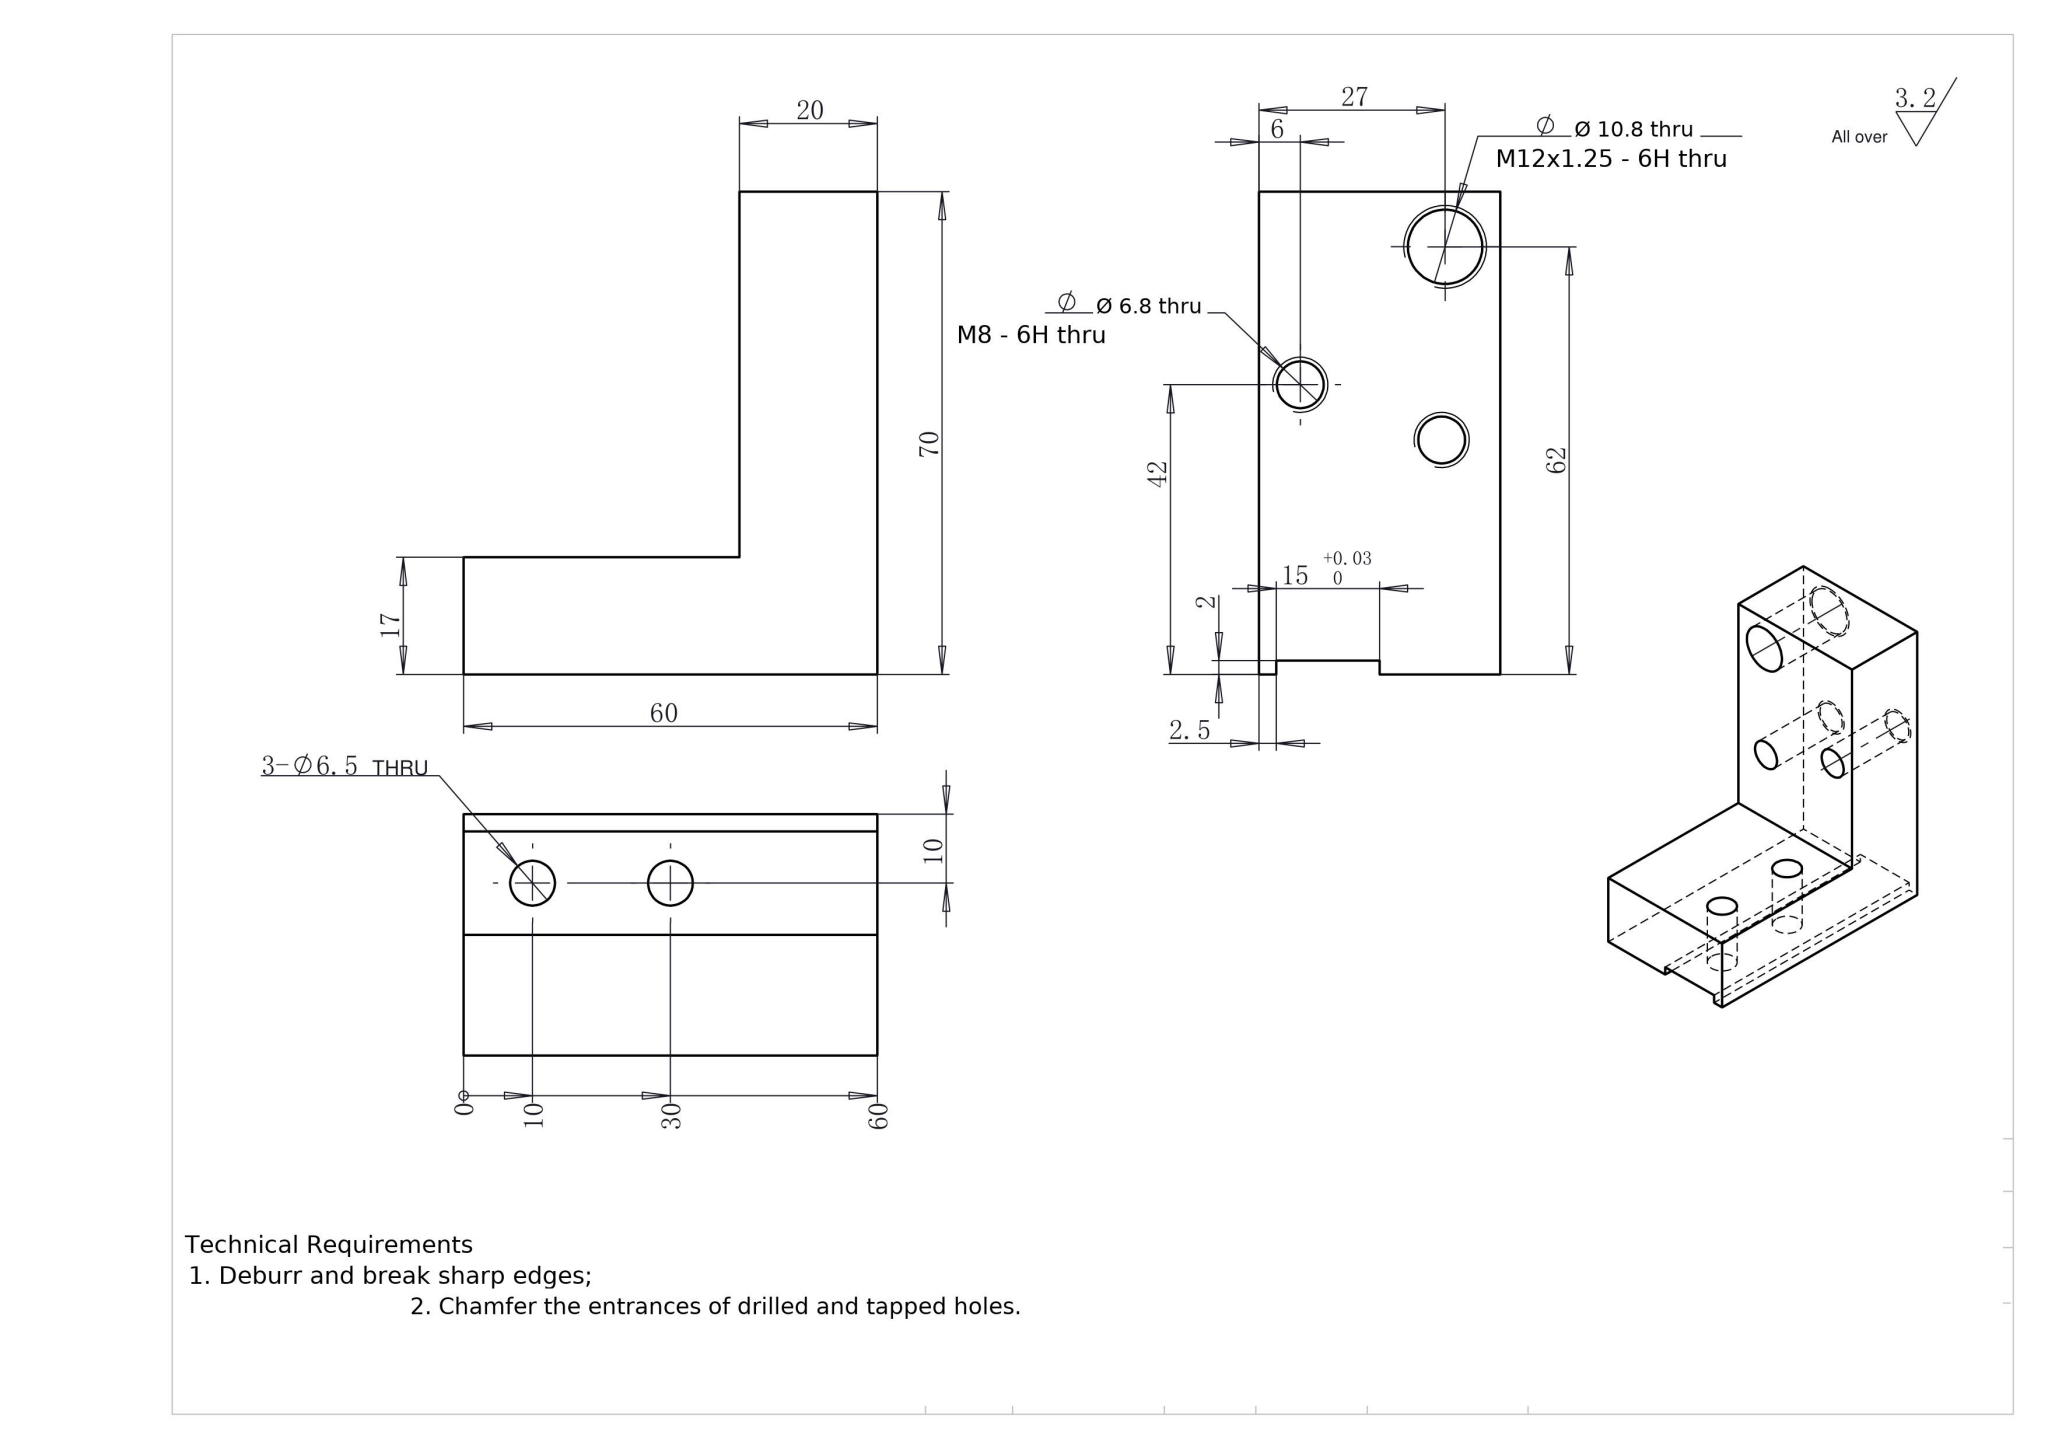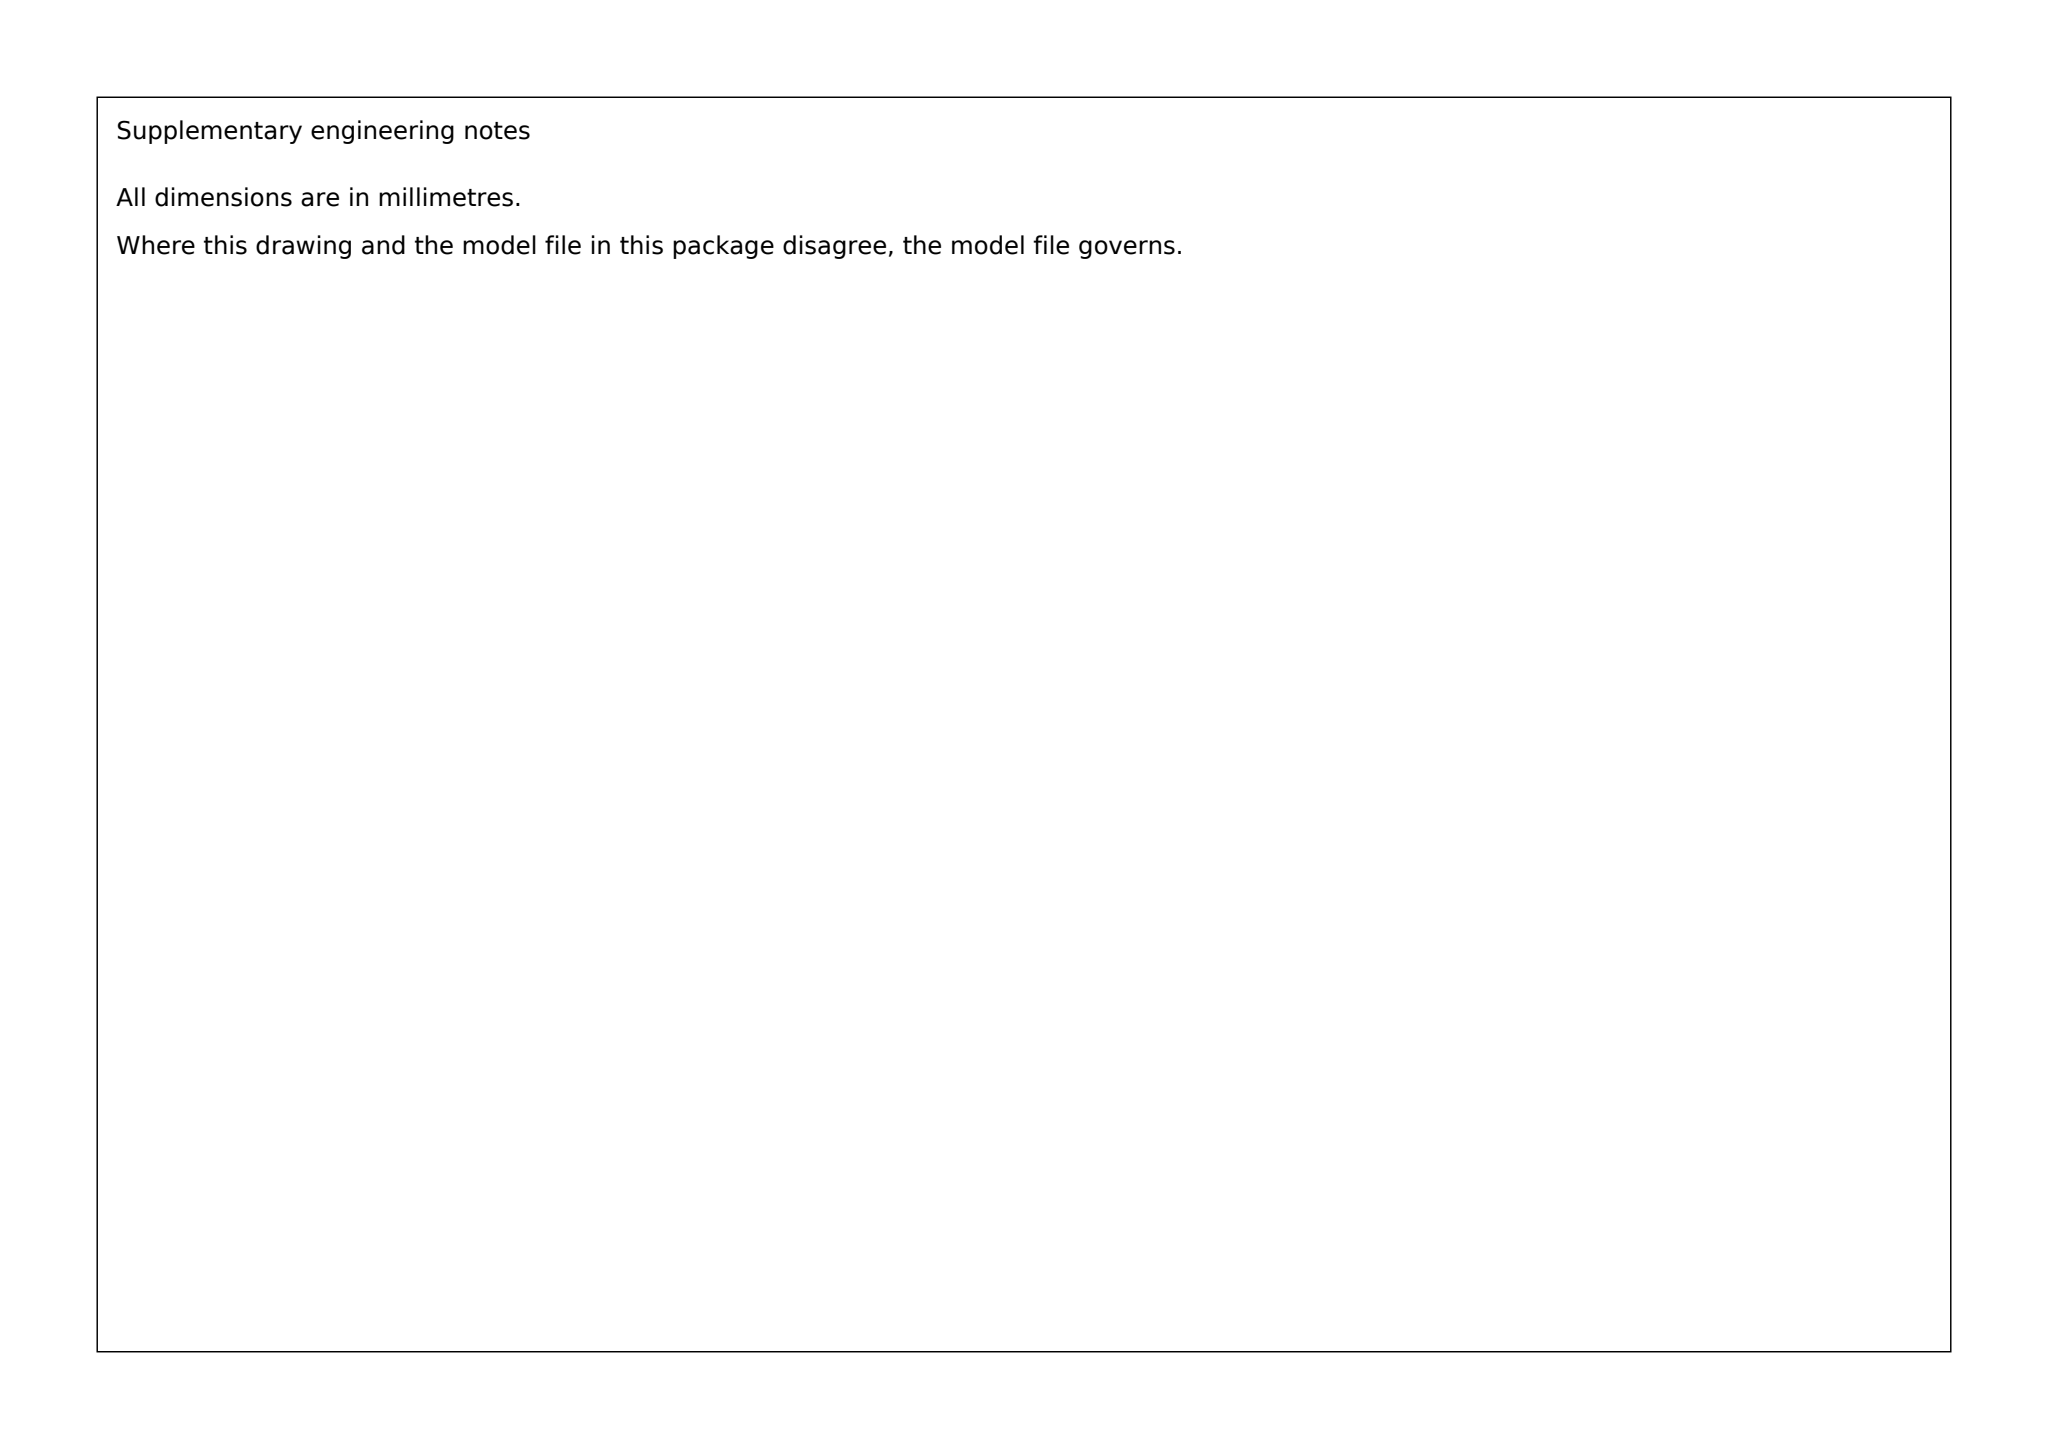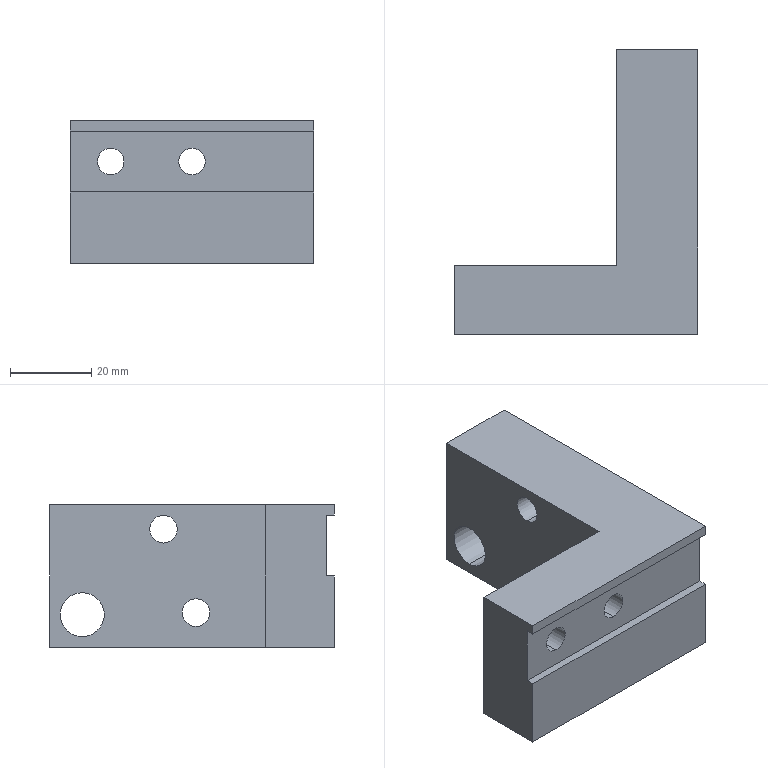Part | SolidWorks | mm | 1 solid | 22 faces | box 60 x 70 x 35 mm | volume 66720 mm3 | plane 12 | cylinder 10 | commonest cylinder face diameters 6.8 x4 6.5 x4 10.8 x2
build123d program:
from build123d import *

# Parameters (mm, degrees)
BOSS_EXTRUDE1_DEPTH     = 35
SKETCH2_W               = 15
SKETCH2_H               = 2
CUT_EXTRUDE1_DEPTH      = 99.615
SKETCH3_R               = 3.25
CUT_EXTRUDE2_DEPTH      = 98.206
M8_TAPPED_HOLE2_D       = 6.8
M12X1_25_TAPPED_HOLE1_D = 10.8
M8_TAPPED_HOLE1_D       = 6.8


with BuildPart() as part:
    # Sketch1 → Boss-Extrude1 (new body)
    with BuildSketch(Plane.XY):
        Polygon((40, 70), (40, 17), (0, 17), (0, 0), (60, 0), (60, 70), align=None)
    extrude(amount=-BOSS_EXTRUDE1_DEPTH)

    # Sketch2 → Cut-Extrude1 (cut, through all)
    with BuildSketch(Plane(origin=(60, 0, 0), x_dir=(0, 0, -1), z_dir=(1, 0, 0))):
        with Locations((10, 1)):
            Rectangle(SKETCH2_W, SKETCH2_H)
    extrude(amount=-CUT_EXTRUDE1_DEPTH, mode=Mode.SUBTRACT)

    # Sketch3 → Cut-Extrude2 (cut, through all)
    with BuildSketch(Plane.XZ.offset(-2)):
        with Locations(Location((10, -10, 0), (0, 0, 270))):
            Circle(SKETCH3_R)
        with Locations(Location((30, -10, 0), (0, 0, 270))):
            Circle(SKETCH3_R)
    extrude(amount=-CUT_EXTRUDE2_DEPTH, mode=Mode.SUBTRACT)

    # M8 Tapped Hole2 (through all)
    with Locations(Plane(origin=(60, 0, 0), x_dir=(0, 0, -1), z_dir=(1, 0, 0))):
        with Locations((6, 42)):
            Hole(M8_TAPPED_HOLE2_D / 2)

    # M12x1.25 Tapped Hole1 (through all)
    with Locations(Plane(origin=(60, 0, 0), x_dir=(0, 0, -1), z_dir=(1, 0, 0))):
        with Locations((27, 62)):
            Hole(M12X1_25_TAPPED_HOLE1_D / 2)

    # M8 Tapped Hole1 (through all)
    with Locations(Plane(origin=(60, 0, 0), x_dir=(0, 0, -1), z_dir=(1, 0, 0))):
        with Locations((26.5, 34)):
            Hole(M8_TAPPED_HOLE1_D / 2)


solid = part.part
STEP:
#1=CARTESIAN_POINT('',(40.,34.,-29.9));
#2=VERTEX_POINT('',#1);
#3=CARTESIAN_POINT('',(40.,34.,-23.1));
#4=VERTEX_POINT('',#3);
#5=CARTESIAN_POINT('',(40.,34.,-26.5));
#6=DIRECTION('',(-1.,0.,0.));
#7=DIRECTION('',(-0.,-1.,0.));
#8=AXIS2_PLACEMENT_3D('',#5,#6,#7);
#9=CIRCLE('',#8,3.4);
#10=EDGE_CURVE('',#2,#4,#9,.T.);
#11=ORIENTED_EDGE('',*,*,#10,.T.);
#12=CARTESIAN_POINT('',(60.,34.,-23.1));
#13=VERTEX_POINT('',#12);
#14=CARTESIAN_POINT('',(60.,34.,-23.1));
#15=DIRECTION('',(1.,0.,0.));
#16=VECTOR('',#15,1000.);
#17=LINE('',#14,#16);
#18=EDGE_CURVE('',#4,#13,#17,.T.);
#19=ORIENTED_EDGE('',*,*,#18,.T.);
#20=CARTESIAN_POINT('',(60.,34.,-29.9));
#21=VERTEX_POINT('',#20);
#22=CARTESIAN_POINT('',(60.,34.,-26.5));
#23=DIRECTION('',(1.,0.,0.));
#24=DIRECTION('',(0.,0.,-1.));
#25=AXIS2_PLACEMENT_3D('',#22,#23,#24);
#26=CIRCLE('',#25,3.4);
#27=EDGE_CURVE('',#13,#21,#26,.T.);
#28=ORIENTED_EDGE('',*,*,#27,.T.);
#29=CARTESIAN_POINT('',(60.,34.,-29.9));
#30=DIRECTION('',(1.,0.,0.));
#31=VECTOR('',#30,1000.);
#32=LINE('',#29,#31);
#33=EDGE_CURVE('',#2,#21,#32,.T.);
#34=ORIENTED_EDGE('',*,*,#33,.F.);
#35=EDGE_LOOP('',(#11,#19,#28,#34));
#36=FACE_OUTER_BOUND('',#35,.T.);
#37=CARTESIAN_POINT('',(60.,34.,-26.5));
#38=DIRECTION('',(1.,0.,0.));
#39=DIRECTION('',(0.,0.,-1.));
#40=AXIS2_PLACEMENT_3D('',#37,#38,#39);
#41=CYLINDRICAL_SURFACE('',#40,3.4);
#42=ADVANCED_FACE('',(#36),#41,.F.);
#43=CARTESIAN_POINT('',(40.,62.,-32.4));
#44=VERTEX_POINT('',#43);
#45=CARTESIAN_POINT('',(40.,62.,-21.6));
#46=VERTEX_POINT('',#45);
#47=CARTESIAN_POINT('',(40.,62.,-27.));
#48=DIRECTION('',(-1.,0.,0.));
#49=DIRECTION('',(-0.,-1.,0.));
#50=AXIS2_PLACEMENT_3D('',#47,#48,#49);
#51=CIRCLE('',#50,5.4);
#52=EDGE_CURVE('',#44,#46,#51,.T.);
#53=ORIENTED_EDGE('',*,*,#52,.T.);
#54=CARTESIAN_POINT('',(60.,62.,-21.6));
#55=VERTEX_POINT('',#54);
#56=CARTESIAN_POINT('',(60.,62.,-21.6));
#57=DIRECTION('',(1.,0.,0.));
#58=VECTOR('',#57,1000.);
#59=LINE('',#56,#58);
#60=EDGE_CURVE('',#46,#55,#59,.T.);
#61=ORIENTED_EDGE('',*,*,#60,.T.);
#62=CARTESIAN_POINT('',(60.,62.,-32.4));
#63=VERTEX_POINT('',#62);
#64=CARTESIAN_POINT('',(60.,62.,-27.));
#65=DIRECTION('',(1.,0.,0.));
#66=DIRECTION('',(0.,0.,-1.));
#67=AXIS2_PLACEMENT_3D('',#64,#65,#66);
#68=CIRCLE('',#67,5.4);
#69=EDGE_CURVE('',#55,#63,#68,.T.);
#70=ORIENTED_EDGE('',*,*,#69,.T.);
#71=CARTESIAN_POINT('',(60.,62.,-32.4));
#72=DIRECTION('',(1.,0.,0.));
#73=VECTOR('',#72,1000.);
#74=LINE('',#71,#73);
#75=EDGE_CURVE('',#44,#63,#74,.T.);
#76=ORIENTED_EDGE('',*,*,#75,.F.);
#77=EDGE_LOOP('',(#53,#61,#70,#76));
#78=FACE_OUTER_BOUND('',#77,.T.);
#79=CARTESIAN_POINT('',(60.,62.,-27.));
#80=DIRECTION('',(1.,0.,0.));
#81=DIRECTION('',(0.,0.,-1.));
#82=AXIS2_PLACEMENT_3D('',#79,#80,#81);
#83=CYLINDRICAL_SURFACE('',#82,5.4);
#84=ADVANCED_FACE('',(#78),#83,.F.);
#85=CARTESIAN_POINT('',(40.,42.,-9.4));
#86=VERTEX_POINT('',#85);
#87=CARTESIAN_POINT('',(40.,42.,-2.6));
#88=VERTEX_POINT('',#87);
#89=CARTESIAN_POINT('',(40.,42.,-6.));
#90=DIRECTION('',(-1.,0.,0.));
#91=DIRECTION('',(-0.,-1.,0.));
#92=AXIS2_PLACEMENT_3D('',#89,#90,#91);
#93=CIRCLE('',#92,3.4);
#94=EDGE_CURVE('',#86,#88,#93,.T.);
#95=ORIENTED_EDGE('',*,*,#94,.T.);
#96=CARTESIAN_POINT('',(60.,42.,-2.6));
#97=VERTEX_POINT('',#96);
#98=CARTESIAN_POINT('',(60.,42.,-2.6));
#99=DIRECTION('',(1.,0.,0.));
#100=VECTOR('',#99,1000.);
#101=LINE('',#98,#100);
#102=EDGE_CURVE('',#88,#97,#101,.T.);
#103=ORIENTED_EDGE('',*,*,#102,.T.);
#104=CARTESIAN_POINT('',(60.,42.,-9.4));
#105=VERTEX_POINT('',#104);
#106=CARTESIAN_POINT('',(60.,42.,-6.));
#107=DIRECTION('',(1.,0.,0.));
#108=DIRECTION('',(0.,0.,-1.));
#109=AXIS2_PLACEMENT_3D('',#106,#107,#108);
#110=CIRCLE('',#109,3.4);
#111=EDGE_CURVE('',#97,#105,#110,.T.);
#112=ORIENTED_EDGE('',*,*,#111,.T.);
#113=CARTESIAN_POINT('',(60.,42.,-9.4));
#114=DIRECTION('',(1.,0.,0.));
#115=VECTOR('',#114,1000.);
#116=LINE('',#113,#115);
#117=EDGE_CURVE('',#86,#105,#116,.T.);
#118=ORIENTED_EDGE('',*,*,#117,.F.);
#119=EDGE_LOOP('',(#95,#103,#112,#118));
#120=FACE_OUTER_BOUND('',#119,.T.);
#121=CARTESIAN_POINT('',(60.,42.,-6.));
#122=DIRECTION('',(1.,0.,0.));
#123=DIRECTION('',(0.,0.,-1.));
#124=AXIS2_PLACEMENT_3D('',#121,#122,#123);
#125=CYLINDRICAL_SURFACE('',#124,3.4);
#126=ADVANCED_FACE('',(#120),#125,.F.);
#127=CARTESIAN_POINT('',(30.,17.,-13.25));
#128=VERTEX_POINT('',#127);
#129=CARTESIAN_POINT('',(30.,17.,-6.75));
#130=VERTEX_POINT('',#129);
#131=CARTESIAN_POINT('',(30.,17.,-10.));
#132=DIRECTION('',(0.,1.,0.));
#133=DIRECTION('',(0.,0.,1.));
#134=AXIS2_PLACEMENT_3D('',#131,#132,#133);
#135=CIRCLE('',#134,3.25);
#136=EDGE_CURVE('',#128,#130,#135,.T.);
#137=ORIENTED_EDGE('',*,*,#136,.T.);
#138=CARTESIAN_POINT('',(30.,2.,-6.75));
#139=VERTEX_POINT('',#138);
#140=CARTESIAN_POINT('',(30.,70.,-6.75));
#141=DIRECTION('',(0.,-1.,-0.));
#142=VECTOR('',#141,1000.);
#143=LINE('',#140,#142);
#144=EDGE_CURVE('',#130,#139,#143,.T.);
#145=ORIENTED_EDGE('',*,*,#144,.T.);
#146=CARTESIAN_POINT('',(30.,2.,-13.25));
#147=VERTEX_POINT('',#146);
#148=CARTESIAN_POINT('',(30.,2.,-10.));
#149=DIRECTION('',(0.,-1.,-0.));
#150=DIRECTION('',(0.,0.,-1.));
#151=AXIS2_PLACEMENT_3D('',#148,#149,#150);
#152=CIRCLE('',#151,3.25);
#153=EDGE_CURVE('',#139,#147,#152,.T.);
#154=ORIENTED_EDGE('',*,*,#153,.T.);
#155=CARTESIAN_POINT('',(30.,70.,-13.25));
#156=DIRECTION('',(0.,-1.,-0.));
#157=VECTOR('',#156,1000.);
#158=LINE('',#155,#157);
#159=EDGE_CURVE('',#128,#147,#158,.T.);
#160=ORIENTED_EDGE('',*,*,#159,.F.);
#161=EDGE_LOOP('',(#137,#145,#154,#160));
#162=FACE_OUTER_BOUND('',#161,.T.);
#163=CARTESIAN_POINT('',(30.,70.,-10.));
#164=DIRECTION('',(0.,-1.,-0.));
#165=DIRECTION('',(0.,0.,-1.));
#166=AXIS2_PLACEMENT_3D('',#163,#164,#165);
#167=CYLINDRICAL_SURFACE('',#166,3.25);
#168=ADVANCED_FACE('',(#162),#167,.F.);
#169=CARTESIAN_POINT('',(10.,17.,-13.25));
#170=VERTEX_POINT('',#169);
#171=CARTESIAN_POINT('',(10.,17.,-6.75));
#172=VERTEX_POINT('',#171);
#173=CARTESIAN_POINT('',(10.,17.,-10.));
#174=DIRECTION('',(0.,1.,0.));
#175=DIRECTION('',(0.,0.,1.));
#176=AXIS2_PLACEMENT_3D('',#173,#174,#175);
#177=CIRCLE('',#176,3.25);
#178=EDGE_CURVE('',#170,#172,#177,.T.);
#179=ORIENTED_EDGE('',*,*,#178,.T.);
#180=CARTESIAN_POINT('',(10.,2.,-6.75));
#181=VERTEX_POINT('',#180);
#182=CARTESIAN_POINT('',(10.,70.,-6.75));
#183=DIRECTION('',(0.,-1.,-0.));
#184=VECTOR('',#183,1000.);
#185=LINE('',#182,#184);
#186=EDGE_CURVE('',#172,#181,#185,.T.);
#187=ORIENTED_EDGE('',*,*,#186,.T.);
#188=CARTESIAN_POINT('',(10.,2.,-13.25));
#189=VERTEX_POINT('',#188);
#190=CARTESIAN_POINT('',(10.,2.,-10.));
#191=DIRECTION('',(0.,-1.,-0.));
#192=DIRECTION('',(0.,0.,-1.));
#193=AXIS2_PLACEMENT_3D('',#190,#191,#192);
#194=CIRCLE('',#193,3.25);
#195=EDGE_CURVE('',#181,#189,#194,.T.);
#196=ORIENTED_EDGE('',*,*,#195,.T.);
#197=CARTESIAN_POINT('',(10.,70.,-13.25));
#198=DIRECTION('',(0.,-1.,-0.));
#199=VECTOR('',#198,1000.);
#200=LINE('',#197,#199);
#201=EDGE_CURVE('',#170,#189,#200,.T.);
#202=ORIENTED_EDGE('',*,*,#201,.F.);
#203=EDGE_LOOP('',(#179,#187,#196,#202));
#204=FACE_OUTER_BOUND('',#203,.T.);
#205=CARTESIAN_POINT('',(10.,70.,-10.));
#206=DIRECTION('',(0.,-1.,-0.));
#207=DIRECTION('',(0.,0.,-1.));
#208=AXIS2_PLACEMENT_3D('',#205,#206,#207);
#209=CYLINDRICAL_SURFACE('',#208,3.25);
#210=ADVANCED_FACE('',(#204),#209,.F.);
#211=CARTESIAN_POINT('',(0.,-0.,-17.5));
#212=VERTEX_POINT('',#211);
#213=CARTESIAN_POINT('',(60.,-0.,-17.5));
#214=VERTEX_POINT('',#213);
#215=CARTESIAN_POINT('',(0.,-0.,-17.5));
#216=DIRECTION('',(1.,0.,0.));
#217=VECTOR('',#216,1000.);
#218=LINE('',#215,#217);
#219=EDGE_CURVE('',#212,#214,#218,.T.);
#220=ORIENTED_EDGE('',*,*,#219,.F.);
#221=CARTESIAN_POINT('',(0.,0.,-35.));
#222=VERTEX_POINT('',#221);
#223=CARTESIAN_POINT('',(0.,0.,-35.));
#224=DIRECTION('',(0.,0.,1.));
#225=VECTOR('',#224,1000.);
#226=LINE('',#223,#225);
#227=EDGE_CURVE('',#222,#212,#226,.T.);
#228=ORIENTED_EDGE('',*,*,#227,.F.);
#229=CARTESIAN_POINT('',(60.,-0.,-35.));
#230=VERTEX_POINT('',#229);
#231=CARTESIAN_POINT('',(0.,0.,-35.));
#232=DIRECTION('',(1.,-0.,0.));
#233=VECTOR('',#232,1000.);
#234=LINE('',#231,#233);
#235=EDGE_CURVE('',#222,#230,#234,.T.);
#236=ORIENTED_EDGE('',*,*,#235,.T.);
#237=CARTESIAN_POINT('',(60.,-0.,-35.));
#238=DIRECTION('',(0.,0.,1.));
#239=VECTOR('',#238,1000.);
#240=LINE('',#237,#239);
#241=EDGE_CURVE('',#230,#214,#240,.T.);
#242=ORIENTED_EDGE('',*,*,#241,.T.);
#243=EDGE_LOOP('',(#220,#228,#236,#242));
#244=FACE_OUTER_BOUND('',#243,.T.);
#245=CARTESIAN_POINT('',(0.,0.,-35.));
#246=DIRECTION('',(-0.,-1.,0.));
#247=DIRECTION('',(1.,-0.,0.));
#248=AXIS2_PLACEMENT_3D('',#245,#246,#247);
#249=PLANE('',#248);
#250=ADVANCED_FACE('',(#244),#249,.T.);
#251=CARTESIAN_POINT('',(60.,70.,0.));
#252=VERTEX_POINT('',#251);
#253=CARTESIAN_POINT('',(40.,70.,0.));
#254=VERTEX_POINT('',#253);
#255=CARTESIAN_POINT('',(40.,70.,0.));
#256=DIRECTION('',(-1.,0.,0.));
#257=VECTOR('',#256,1000.);
#258=LINE('',#255,#257);
#259=EDGE_CURVE('',#252,#254,#258,.T.);
#260=ORIENTED_EDGE('',*,*,#259,.F.);
#261=CARTESIAN_POINT('',(60.,70.,-35.));
#262=VERTEX_POINT('',#261);
#263=CARTESIAN_POINT('',(60.,70.,-35.));
#264=DIRECTION('',(0.,0.,1.));
#265=VECTOR('',#264,1000.);
#266=LINE('',#263,#265);
#267=EDGE_CURVE('',#262,#252,#266,.T.);
#268=ORIENTED_EDGE('',*,*,#267,.F.);
#269=CARTESIAN_POINT('',(40.,70.,-35.));
#270=VERTEX_POINT('',#269);
#271=CARTESIAN_POINT('',(40.,70.,-35.));
#272=DIRECTION('',(-1.,0.,0.));
#273=VECTOR('',#272,1000.);
#274=LINE('',#271,#273);
#275=EDGE_CURVE('',#262,#270,#274,.T.);
#276=ORIENTED_EDGE('',*,*,#275,.T.);
#277=CARTESIAN_POINT('',(40.,70.,-35.));
#278=DIRECTION('',(0.,0.,1.));
#279=VECTOR('',#278,1000.);
#280=LINE('',#277,#279);
#281=EDGE_CURVE('',#270,#254,#280,.T.);
#282=ORIENTED_EDGE('',*,*,#281,.T.);
#283=EDGE_LOOP('',(#260,#268,#276,#282));
#284=FACE_OUTER_BOUND('',#283,.T.);
#285=CARTESIAN_POINT('',(40.,70.,-35.));
#286=DIRECTION('',(0.,1.,0.));
#287=DIRECTION('',(0.,0.,1.));
#288=AXIS2_PLACEMENT_3D('',#285,#286,#287);
#289=PLANE('',#288);
#290=ADVANCED_FACE('',(#284),#289,.T.);
#291=CARTESIAN_POINT('',(60.,34.,-26.5));
#292=DIRECTION('',(1.,0.,0.));
#293=DIRECTION('',(0.,0.,-1.));
#294=AXIS2_PLACEMENT_3D('',#291,#292,#293);
#295=CIRCLE('',#294,3.4);
#296=EDGE_CURVE('',#21,#13,#295,.T.);
#297=ORIENTED_EDGE('',*,*,#296,.F.);
#298=ORIENTED_EDGE('',*,*,#27,.F.);
#299=EDGE_LOOP('',(#297,#298));
#300=FACE_BOUND('',#299,.T.);
#301=CARTESIAN_POINT('',(60.,62.,-27.));
#302=DIRECTION('',(1.,0.,0.));
#303=DIRECTION('',(0.,0.,-1.));
#304=AXIS2_PLACEMENT_3D('',#301,#302,#303);
#305=CIRCLE('',#304,5.4);
#306=EDGE_CURVE('',#63,#55,#305,.T.);
#307=ORIENTED_EDGE('',*,*,#306,.F.);
#308=ORIENTED_EDGE('',*,*,#69,.F.);
#309=EDGE_LOOP('',(#307,#308));
#310=FACE_BOUND('',#309,.T.);
#311=CARTESIAN_POINT('',(60.,42.,-6.));
#312=DIRECTION('',(1.,0.,0.));
#313=DIRECTION('',(0.,0.,-1.));
#314=AXIS2_PLACEMENT_3D('',#311,#312,#313);
#315=CIRCLE('',#314,3.4);
#316=EDGE_CURVE('',#105,#97,#315,.T.);
#317=ORIENTED_EDGE('',*,*,#316,.F.);
#318=ORIENTED_EDGE('',*,*,#111,.F.);
#319=EDGE_LOOP('',(#317,#318));
#320=FACE_BOUND('',#319,.T.);
#321=CARTESIAN_POINT('',(60.,2.,-17.5));
#322=VERTEX_POINT('',#321);
#323=CARTESIAN_POINT('',(60.,-0.,-17.5));
#324=DIRECTION('',(0.,1.,0.));
#325=VECTOR('',#324,1000.);
#326=LINE('',#323,#325);
#327=EDGE_CURVE('',#214,#322,#326,.T.);
#328=ORIENTED_EDGE('',*,*,#327,.F.);
#329=ORIENTED_EDGE('',*,*,#241,.F.);
#330=CARTESIAN_POINT('',(60.,70.,-35.));
#331=DIRECTION('',(0.,1.,0.));
#332=VECTOR('',#331,1000.);
#333=LINE('',#330,#332);
#334=EDGE_CURVE('',#230,#262,#333,.T.);
#335=ORIENTED_EDGE('',*,*,#334,.T.);
#336=ORIENTED_EDGE('',*,*,#267,.T.);
#337=CARTESIAN_POINT('',(60.,-0.,0.));
#338=VERTEX_POINT('',#337);
#339=CARTESIAN_POINT('',(60.,70.,0.));
#340=DIRECTION('',(0.,1.,0.));
#341=VECTOR('',#340,1000.);
#342=LINE('',#339,#341);
#343=EDGE_CURVE('',#338,#252,#342,.T.);
#344=ORIENTED_EDGE('',*,*,#343,.F.);
#345=CARTESIAN_POINT('',(60.,-0.,-2.5));
#346=VERTEX_POINT('',#345);
#347=CARTESIAN_POINT('',(60.,-0.,-35.));
#348=DIRECTION('',(0.,0.,1.));
#349=VECTOR('',#348,1000.);
#350=LINE('',#347,#349);
#351=EDGE_CURVE('',#346,#338,#350,.T.);
#352=ORIENTED_EDGE('',*,*,#351,.F.);
#353=CARTESIAN_POINT('',(60.,2.,-2.5));
#354=VERTEX_POINT('',#353);
#355=CARTESIAN_POINT('',(60.,-0.,-2.5));
#356=DIRECTION('',(0.,-1.,0.));
#357=VECTOR('',#356,1000.);
#358=LINE('',#355,#357);
#359=EDGE_CURVE('',#354,#346,#358,.T.);
#360=ORIENTED_EDGE('',*,*,#359,.F.);
#361=CARTESIAN_POINT('',(60.,2.,-17.5));
#362=DIRECTION('',(0.,-0.,1.));
#363=VECTOR('',#362,1000.);
#364=LINE('',#361,#363);
#365=EDGE_CURVE('',#322,#354,#364,.T.);
#366=ORIENTED_EDGE('',*,*,#365,.F.);
#367=EDGE_LOOP('',(#328,#329,#335,#336,#344,#352,#360,#366));
#368=FACE_OUTER_BOUND('',#367,.T.);
#369=CARTESIAN_POINT('',(60.,70.,-35.));
#370=DIRECTION('',(1.,-0.,0.));
#371=DIRECTION('',(0.,1.,0.));
#372=AXIS2_PLACEMENT_3D('',#369,#370,#371);
#373=PLANE('',#372);
#374=ADVANCED_FACE('',(#300,#310,#320,#368),#373,.T.);
#375=CARTESIAN_POINT('',(0.,-0.,-2.5));
#376=VERTEX_POINT('',#375);
#377=CARTESIAN_POINT('',(0.,-0.,-2.5));
#378=DIRECTION('',(1.,0.,0.));
#379=VECTOR('',#378,1000.);
#380=LINE('',#377,#379);
#381=EDGE_CURVE('',#376,#346,#380,.T.);
#382=ORIENTED_EDGE('',*,*,#381,.T.);
#383=ORIENTED_EDGE('',*,*,#351,.T.);
#384=CARTESIAN_POINT('',(0.,0.,0.));
#385=VERTEX_POINT('',#384);
#386=CARTESIAN_POINT('',(0.,0.,0.));
#387=DIRECTION('',(1.,-0.,0.));
#388=VECTOR('',#387,1000.);
#389=LINE('',#386,#388);
#390=EDGE_CURVE('',#385,#338,#389,.T.);
#391=ORIENTED_EDGE('',*,*,#390,.F.);
#392=CARTESIAN_POINT('',(0.,0.,-35.));
#393=DIRECTION('',(0.,0.,1.));
#394=VECTOR('',#393,1000.);
#395=LINE('',#392,#394);
#396=EDGE_CURVE('',#376,#385,#395,.T.);
#397=ORIENTED_EDGE('',*,*,#396,.F.);
#398=EDGE_LOOP('',(#382,#383,#391,#397));
#399=FACE_OUTER_BOUND('',#398,.T.);
#400=CARTESIAN_POINT('',(0.,0.,-35.));
#401=DIRECTION('',(-0.,-1.,0.));
#402=DIRECTION('',(1.,-0.,0.));
#403=AXIS2_PLACEMENT_3D('',#400,#401,#402);
#404=PLANE('',#403);
#405=ADVANCED_FACE('',(#399),#404,.T.);
#406=CARTESIAN_POINT('',(0.,2.,-17.5));
#407=VERTEX_POINT('',#406);
#408=CARTESIAN_POINT('',(0.,-0.,-17.5));
#409=DIRECTION('',(0.,1.,0.));
#410=VECTOR('',#409,1000.);
#411=LINE('',#408,#410);
#412=EDGE_CURVE('',#212,#407,#411,.T.);
#413=ORIENTED_EDGE('',*,*,#412,.T.);
#414=CARTESIAN_POINT('',(0.,2.,-2.5));
#415=VERTEX_POINT('',#414);
#416=CARTESIAN_POINT('',(0.,2.,-17.5));
#417=DIRECTION('',(0.,-0.,1.));
#418=VECTOR('',#417,1000.);
#419=LINE('',#416,#418);
#420=EDGE_CURVE('',#407,#415,#419,.T.);
#421=ORIENTED_EDGE('',*,*,#420,.T.);
#422=CARTESIAN_POINT('',(0.,-0.,-2.5));
#423=DIRECTION('',(0.,-1.,0.));
#424=VECTOR('',#423,1000.);
#425=LINE('',#422,#424);
#426=EDGE_CURVE('',#415,#376,#425,.T.);
#427=ORIENTED_EDGE('',*,*,#426,.T.);
#428=ORIENTED_EDGE('',*,*,#396,.T.);
#429=CARTESIAN_POINT('',(0.,17.,0.));
#430=VERTEX_POINT('',#429);
#431=CARTESIAN_POINT('',(0.,17.,0.));
#432=DIRECTION('',(-0.,-1.,0.));
#433=VECTOR('',#432,1000.);
#434=LINE('',#431,#433);
#435=EDGE_CURVE('',#430,#385,#434,.T.);
#436=ORIENTED_EDGE('',*,*,#435,.F.);
#437=CARTESIAN_POINT('',(0.,17.,-35.));
#438=VERTEX_POINT('',#437);
#439=CARTESIAN_POINT('',(0.,17.,-35.));
#440=DIRECTION('',(0.,0.,1.));
#441=VECTOR('',#440,1000.);
#442=LINE('',#439,#441);
#443=EDGE_CURVE('',#438,#430,#442,.T.);
#444=ORIENTED_EDGE('',*,*,#443,.F.);
#445=CARTESIAN_POINT('',(0.,17.,-35.));
#446=DIRECTION('',(-0.,-1.,0.));
#447=VECTOR('',#446,1000.);
#448=LINE('',#445,#447);
#449=EDGE_CURVE('',#438,#222,#448,.T.);
#450=ORIENTED_EDGE('',*,*,#449,.T.);
#451=ORIENTED_EDGE('',*,*,#227,.T.);
#452=EDGE_LOOP('',(#413,#421,#427,#428,#436,#444,#450,#451));
#453=FACE_OUTER_BOUND('',#452,.T.);
#454=CARTESIAN_POINT('',(0.,17.,-35.));
#455=DIRECTION('',(-1.,0.,0.));
#456=DIRECTION('',(-0.,-1.,0.));
#457=AXIS2_PLACEMENT_3D('',#454,#455,#456);
#458=PLANE('',#457);
#459=ADVANCED_FACE('',(#453),#458,.T.);
#460=ORIENTED_EDGE('',*,*,#136,.F.);
#461=CARTESIAN_POINT('',(30.,17.,-10.));
#462=DIRECTION('',(0.,1.,0.));
#463=DIRECTION('',(0.,0.,1.));
#464=AXIS2_PLACEMENT_3D('',#461,#462,#463);
#465=CIRCLE('',#464,3.25);
#466=EDGE_CURVE('',#130,#128,#465,.T.);
#467=ORIENTED_EDGE('',*,*,#466,.F.);
#468=EDGE_LOOP('',(#460,#467));
#469=FACE_BOUND('',#468,.T.);
#470=ORIENTED_EDGE('',*,*,#178,.F.);
#471=CARTESIAN_POINT('',(10.,17.,-10.));
#472=DIRECTION('',(0.,1.,0.));
#473=DIRECTION('',(0.,0.,1.));
#474=AXIS2_PLACEMENT_3D('',#471,#472,#473);
#475=CIRCLE('',#474,3.25);
#476=EDGE_CURVE('',#172,#170,#475,.T.);
#477=ORIENTED_EDGE('',*,*,#476,.F.);
#478=EDGE_LOOP('',(#470,#477));
#479=FACE_BOUND('',#478,.T.);
#480=CARTESIAN_POINT('',(40.,17.,0.));
#481=VERTEX_POINT('',#480);
#482=CARTESIAN_POINT('',(0.,17.,0.));
#483=DIRECTION('',(-1.,0.,0.));
#484=VECTOR('',#483,1000.);
#485=LINE('',#482,#484);
#486=EDGE_CURVE('',#481,#430,#485,.T.);
#487=ORIENTED_EDGE('',*,*,#486,.F.);
#488=CARTESIAN_POINT('',(40.,17.,-35.));
#489=VERTEX_POINT('',#488);
#490=CARTESIAN_POINT('',(40.,17.,-35.));
#491=DIRECTION('',(0.,0.,1.));
#492=VECTOR('',#491,1000.);
#493=LINE('',#490,#492);
#494=EDGE_CURVE('',#489,#481,#493,.T.);
#495=ORIENTED_EDGE('',*,*,#494,.F.);
#496=CARTESIAN_POINT('',(0.,17.,-35.));
#497=DIRECTION('',(-1.,0.,0.));
#498=VECTOR('',#497,1000.);
#499=LINE('',#496,#498);
#500=EDGE_CURVE('',#489,#438,#499,.T.);
#501=ORIENTED_EDGE('',*,*,#500,.T.);
#502=ORIENTED_EDGE('',*,*,#443,.T.);
#503=EDGE_LOOP('',(#487,#495,#501,#502));
#504=FACE_OUTER_BOUND('',#503,.T.);
#505=CARTESIAN_POINT('',(0.,17.,-35.));
#506=DIRECTION('',(0.,1.,0.));
#507=DIRECTION('',(0.,0.,1.));
#508=AXIS2_PLACEMENT_3D('',#505,#506,#507);
#509=PLANE('',#508);
#510=ADVANCED_FACE('',(#469,#479,#504),#509,.T.);
#511=ORIENTED_EDGE('',*,*,#10,.F.);
#512=CARTESIAN_POINT('',(40.,34.,-26.5));
#513=DIRECTION('',(-1.,0.,0.));
#514=DIRECTION('',(-0.,-1.,0.));
#515=AXIS2_PLACEMENT_3D('',#512,#513,#514);
#516=CIRCLE('',#515,3.4);
#517=EDGE_CURVE('',#4,#2,#516,.T.);
#518=ORIENTED_EDGE('',*,*,#517,.F.);
#519=EDGE_LOOP('',(#511,#518));
#520=FACE_BOUND('',#519,.T.);
#521=ORIENTED_EDGE('',*,*,#52,.F.);
#522=CARTESIAN_POINT('',(40.,62.,-27.));
#523=DIRECTION('',(-1.,0.,0.));
#524=DIRECTION('',(-0.,-1.,0.));
#525=AXIS2_PLACEMENT_3D('',#522,#523,#524);
#526=CIRCLE('',#525,5.4);
#527=EDGE_CURVE('',#46,#44,#526,.T.);
#528=ORIENTED_EDGE('',*,*,#527,.F.);
#529=EDGE_LOOP('',(#521,#528));
#530=FACE_BOUND('',#529,.T.);
#531=ORIENTED_EDGE('',*,*,#94,.F.);
#532=CARTESIAN_POINT('',(40.,42.,-6.));
#533=DIRECTION('',(-1.,0.,0.));
#534=DIRECTION('',(-0.,-1.,0.));
#535=AXIS2_PLACEMENT_3D('',#532,#533,#534);
#536=CIRCLE('',#535,3.4);
#537=EDGE_CURVE('',#88,#86,#536,.T.);
#538=ORIENTED_EDGE('',*,*,#537,.F.);
#539=EDGE_LOOP('',(#531,#538));
#540=FACE_BOUND('',#539,.T.);
#541=CARTESIAN_POINT('',(40.,70.,0.));
#542=DIRECTION('',(-0.,-1.,0.));
#543=VECTOR('',#542,1000.);
#544=LINE('',#541,#543);
#545=EDGE_CURVE('',#254,#481,#544,.T.);
#546=ORIENTED_EDGE('',*,*,#545,.F.);
#547=ORIENTED_EDGE('',*,*,#281,.F.);
#548=CARTESIAN_POINT('',(40.,70.,-35.));
#549=DIRECTION('',(-0.,-1.,0.));
#550=VECTOR('',#549,1000.);
#551=LINE('',#548,#550);
#552=EDGE_CURVE('',#270,#489,#551,.T.);
#553=ORIENTED_EDGE('',*,*,#552,.T.);
#554=ORIENTED_EDGE('',*,*,#494,.T.);
#555=EDGE_LOOP('',(#546,#547,#553,#554));
#556=FACE_OUTER_BOUND('',#555,.T.);
#557=CARTESIAN_POINT('',(40.,70.,-35.));
#558=DIRECTION('',(-1.,0.,0.));
#559=DIRECTION('',(-0.,-1.,0.));
#560=AXIS2_PLACEMENT_3D('',#557,#558,#559);
#561=PLANE('',#560);
#562=ADVANCED_FACE('',(#520,#530,#540,#556),#561,.T.);
#563=ORIENTED_EDGE('',*,*,#275,.F.);
#564=ORIENTED_EDGE('',*,*,#334,.F.);
#565=ORIENTED_EDGE('',*,*,#235,.F.);
#566=ORIENTED_EDGE('',*,*,#449,.F.);
#567=ORIENTED_EDGE('',*,*,#500,.F.);
#568=ORIENTED_EDGE('',*,*,#552,.F.);
#569=EDGE_LOOP('',(#563,#564,#565,#566,#567,#568));
#570=FACE_OUTER_BOUND('',#569,.T.);
#571=CARTESIAN_POINT('',(0.,0.,-35.));
#572=DIRECTION('',(0.,0.,-1.));
#573=DIRECTION('',(-1.,0.,0.));
#574=AXIS2_PLACEMENT_3D('',#571,#572,#573);
#575=PLANE('',#574);
#576=ADVANCED_FACE('',(#570),#575,.T.);
#577=ORIENTED_EDGE('',*,*,#259,.T.);
#578=ORIENTED_EDGE('',*,*,#545,.T.);
#579=ORIENTED_EDGE('',*,*,#486,.T.);
#580=ORIENTED_EDGE('',*,*,#435,.T.);
#581=ORIENTED_EDGE('',*,*,#390,.T.);
#582=ORIENTED_EDGE('',*,*,#343,.T.);
#583=EDGE_LOOP('',(#577,#578,#579,#580,#581,#582));
#584=FACE_OUTER_BOUND('',#583,.T.);
#585=CARTESIAN_POINT('',(0.,0.,0.));
#586=DIRECTION('',(0.,0.,-1.));
#587=DIRECTION('',(-1.,0.,0.));
#588=AXIS2_PLACEMENT_3D('',#585,#586,#587);
#589=PLANE('',#588);
#590=ADVANCED_FACE('',(#584),#589,.F.);
#591=ORIENTED_EDGE('',*,*,#327,.T.);
#592=CARTESIAN_POINT('',(0.,2.,-17.5));
#593=DIRECTION('',(1.,0.,0.));
#594=VECTOR('',#593,1000.);
#595=LINE('',#592,#594);
#596=EDGE_CURVE('',#407,#322,#595,.T.);
#597=ORIENTED_EDGE('',*,*,#596,.F.);
#598=ORIENTED_EDGE('',*,*,#412,.F.);
#599=ORIENTED_EDGE('',*,*,#219,.T.);
#600=EDGE_LOOP('',(#591,#597,#598,#599));
#601=FACE_OUTER_BOUND('',#600,.T.);
#602=CARTESIAN_POINT('',(0.,-0.,-17.5));
#603=DIRECTION('',(0.,0.,-1.));
#604=DIRECTION('',(-1.,0.,0.));
#605=AXIS2_PLACEMENT_3D('',#602,#603,#604);
#606=PLANE('',#605);
#607=ADVANCED_FACE('',(#601),#606,.F.);
#608=ORIENTED_EDGE('',*,*,#359,.T.);
#609=ORIENTED_EDGE('',*,*,#381,.F.);
#610=ORIENTED_EDGE('',*,*,#426,.F.);
#611=CARTESIAN_POINT('',(0.,2.,-2.5));
#612=DIRECTION('',(1.,0.,0.));
#613=VECTOR('',#612,1000.);
#614=LINE('',#611,#613);
#615=EDGE_CURVE('',#415,#354,#614,.T.);
#616=ORIENTED_EDGE('',*,*,#615,.T.);
#617=EDGE_LOOP('',(#608,#609,#610,#616));
#618=FACE_OUTER_BOUND('',#617,.T.);
#619=CARTESIAN_POINT('',(0.,-0.,-2.5));
#620=DIRECTION('',(0.,0.,1.));
#621=DIRECTION('',(0.,-1.,0.));
#622=AXIS2_PLACEMENT_3D('',#619,#620,#621);
#623=PLANE('',#622);
#624=ADVANCED_FACE('',(#618),#623,.F.);
#625=CARTESIAN_POINT('',(30.,2.,-10.));
#626=DIRECTION('',(0.,-1.,-0.));
#627=DIRECTION('',(0.,0.,-1.));
#628=AXIS2_PLACEMENT_3D('',#625,#626,#627);
#629=CIRCLE('',#628,3.25);
#630=EDGE_CURVE('',#147,#139,#629,.T.);
#631=ORIENTED_EDGE('',*,*,#630,.F.);
#632=ORIENTED_EDGE('',*,*,#153,.F.);
#633=EDGE_LOOP('',(#631,#632));
#634=FACE_BOUND('',#633,.T.);
#635=CARTESIAN_POINT('',(10.,2.,-10.));
#636=DIRECTION('',(0.,-1.,-0.));
#637=DIRECTION('',(0.,0.,-1.));
#638=AXIS2_PLACEMENT_3D('',#635,#636,#637);
#639=CIRCLE('',#638,3.25);
#640=EDGE_CURVE('',#189,#181,#639,.T.);
#641=ORIENTED_EDGE('',*,*,#640,.F.);
#642=ORIENTED_EDGE('',*,*,#195,.F.);
#643=EDGE_LOOP('',(#641,#642));
#644=FACE_BOUND('',#643,.T.);
#645=ORIENTED_EDGE('',*,*,#365,.T.);
#646=ORIENTED_EDGE('',*,*,#615,.F.);
#647=ORIENTED_EDGE('',*,*,#420,.F.);
#648=ORIENTED_EDGE('',*,*,#596,.T.);
#649=EDGE_LOOP('',(#645,#646,#647,#648));
#650=FACE_OUTER_BOUND('',#649,.T.);
#651=CARTESIAN_POINT('',(0.,2.,-17.5));
#652=DIRECTION('',(0.,1.,0.));
#653=DIRECTION('',(0.,-0.,1.));
#654=AXIS2_PLACEMENT_3D('',#651,#652,#653);
#655=PLANE('',#654);
#656=ADVANCED_FACE('',(#634,#644,#650),#655,.F.);
#657=ORIENTED_EDGE('',*,*,#186,.F.);
#658=ORIENTED_EDGE('',*,*,#476,.T.);
#659=ORIENTED_EDGE('',*,*,#201,.T.);
#660=ORIENTED_EDGE('',*,*,#640,.T.);
#661=EDGE_LOOP('',(#657,#658,#659,#660));
#662=FACE_OUTER_BOUND('',#661,.T.);
#663=CARTESIAN_POINT('',(10.,70.,-10.));
#664=DIRECTION('',(0.,-1.,-0.));
#665=DIRECTION('',(0.,0.,-1.));
#666=AXIS2_PLACEMENT_3D('',#663,#664,#665);
#667=CYLINDRICAL_SURFACE('',#666,3.25);
#668=ADVANCED_FACE('',(#662),#667,.F.);
#669=ORIENTED_EDGE('',*,*,#144,.F.);
#670=ORIENTED_EDGE('',*,*,#466,.T.);
#671=ORIENTED_EDGE('',*,*,#159,.T.);
#672=ORIENTED_EDGE('',*,*,#630,.T.);
#673=EDGE_LOOP('',(#669,#670,#671,#672));
#674=FACE_OUTER_BOUND('',#673,.T.);
#675=CARTESIAN_POINT('',(30.,70.,-10.));
#676=DIRECTION('',(0.,-1.,-0.));
#677=DIRECTION('',(0.,0.,-1.));
#678=AXIS2_PLACEMENT_3D('',#675,#676,#677);
#679=CYLINDRICAL_SURFACE('',#678,3.25);
#680=ADVANCED_FACE('',(#674),#679,.F.);
#681=ORIENTED_EDGE('',*,*,#102,.F.);
#682=ORIENTED_EDGE('',*,*,#537,.T.);
#683=ORIENTED_EDGE('',*,*,#117,.T.);
#684=ORIENTED_EDGE('',*,*,#316,.T.);
#685=EDGE_LOOP('',(#681,#682,#683,#684));
#686=FACE_OUTER_BOUND('',#685,.T.);
#687=CARTESIAN_POINT('',(60.,42.,-6.));
#688=DIRECTION('',(1.,0.,0.));
#689=DIRECTION('',(0.,0.,-1.));
#690=AXIS2_PLACEMENT_3D('',#687,#688,#689);
#691=CYLINDRICAL_SURFACE('',#690,3.4);
#692=ADVANCED_FACE('',(#686),#691,.F.);
#693=ORIENTED_EDGE('',*,*,#60,.F.);
#694=ORIENTED_EDGE('',*,*,#527,.T.);
#695=ORIENTED_EDGE('',*,*,#75,.T.);
#696=ORIENTED_EDGE('',*,*,#306,.T.);
#697=EDGE_LOOP('',(#693,#694,#695,#696));
#698=FACE_OUTER_BOUND('',#697,.T.);
#699=CARTESIAN_POINT('',(60.,62.,-27.));
#700=DIRECTION('',(1.,0.,0.));
#701=DIRECTION('',(0.,0.,-1.));
#702=AXIS2_PLACEMENT_3D('',#699,#700,#701);
#703=CYLINDRICAL_SURFACE('',#702,5.4);
#704=ADVANCED_FACE('',(#698),#703,.F.);
#705=ORIENTED_EDGE('',*,*,#18,.F.);
#706=ORIENTED_EDGE('',*,*,#517,.T.);
#707=ORIENTED_EDGE('',*,*,#33,.T.);
#708=ORIENTED_EDGE('',*,*,#296,.T.);
#709=EDGE_LOOP('',(#705,#706,#707,#708));
#710=FACE_OUTER_BOUND('',#709,.T.);
#711=CARTESIAN_POINT('',(60.,34.,-26.5));
#712=DIRECTION('',(1.,0.,0.));
#713=DIRECTION('',(0.,0.,-1.));
#714=AXIS2_PLACEMENT_3D('',#711,#712,#713);
#715=CYLINDRICAL_SURFACE('',#714,3.4);
#716=ADVANCED_FACE('',(#710),#715,.F.);
#717=CLOSED_SHELL('',(#42,#84,#126,#168,#210,#250,#290,#374,#405,#459,#510,#562,#576,#590,#607,#624,#656,#668,#680,#692,#704,#716));
#718=MANIFOLD_SOLID_BREP('',#717);
#719=CARTESIAN_POINT('',(0.,0.,0.));
#720=DIRECTION('',(0.,0.,1.));
#721=DIRECTION('',(1.,0.,0.));
#722=AXIS2_PLACEMENT_3D('',#719,#720,#721);
#723=(LENGTH_UNIT()NAMED_UNIT(*)SI_UNIT(.MILLI.,.METRE.));
#724=UNCERTAINTY_MEASURE_WITH_UNIT(LENGTH_MEASURE(0.00001),#723,'','');
#725=(NAMED_UNIT(*)PLANE_ANGLE_UNIT()SI_UNIT($,.RADIAN.));
#726=(NAMED_UNIT(*)SI_UNIT($,.STERADIAN.)SOLID_ANGLE_UNIT());
#727=(GEOMETRIC_REPRESENTATION_CONTEXT(3)GLOBAL_UNCERTAINTY_ASSIGNED_CONTEXT((#724))GLOBAL_UNIT_ASSIGNED_CONTEXT((#723,#725,#726))REPRESENTATION_CONTEXT('',''));
#728=ADVANCED_BREP_SHAPE_REPRESENTATION('',(#718,#722),#727);